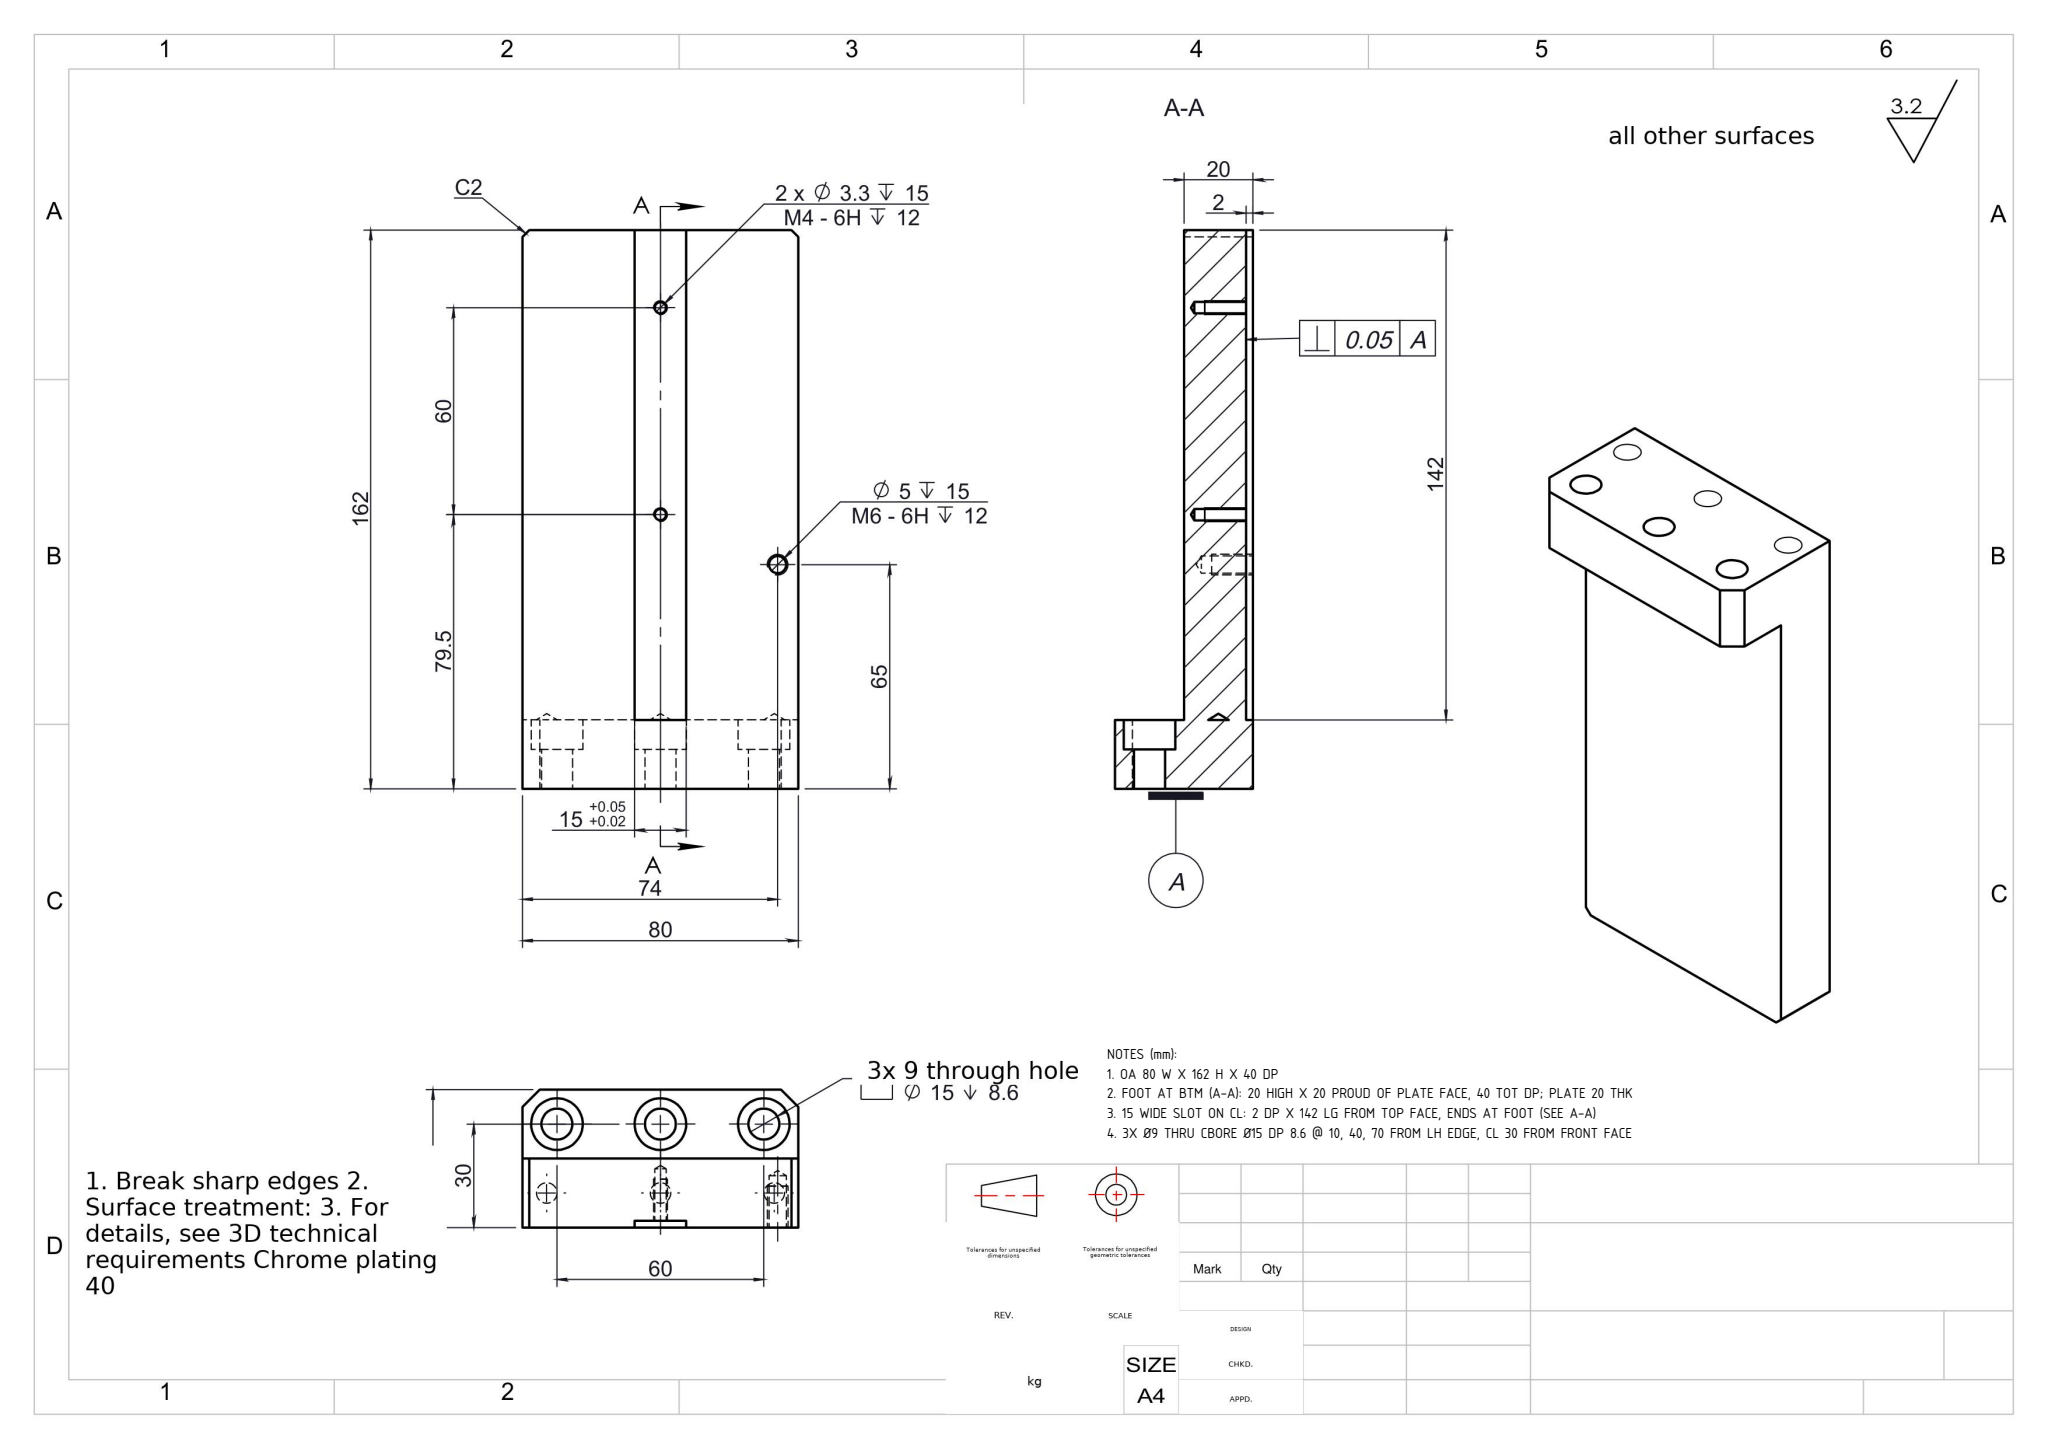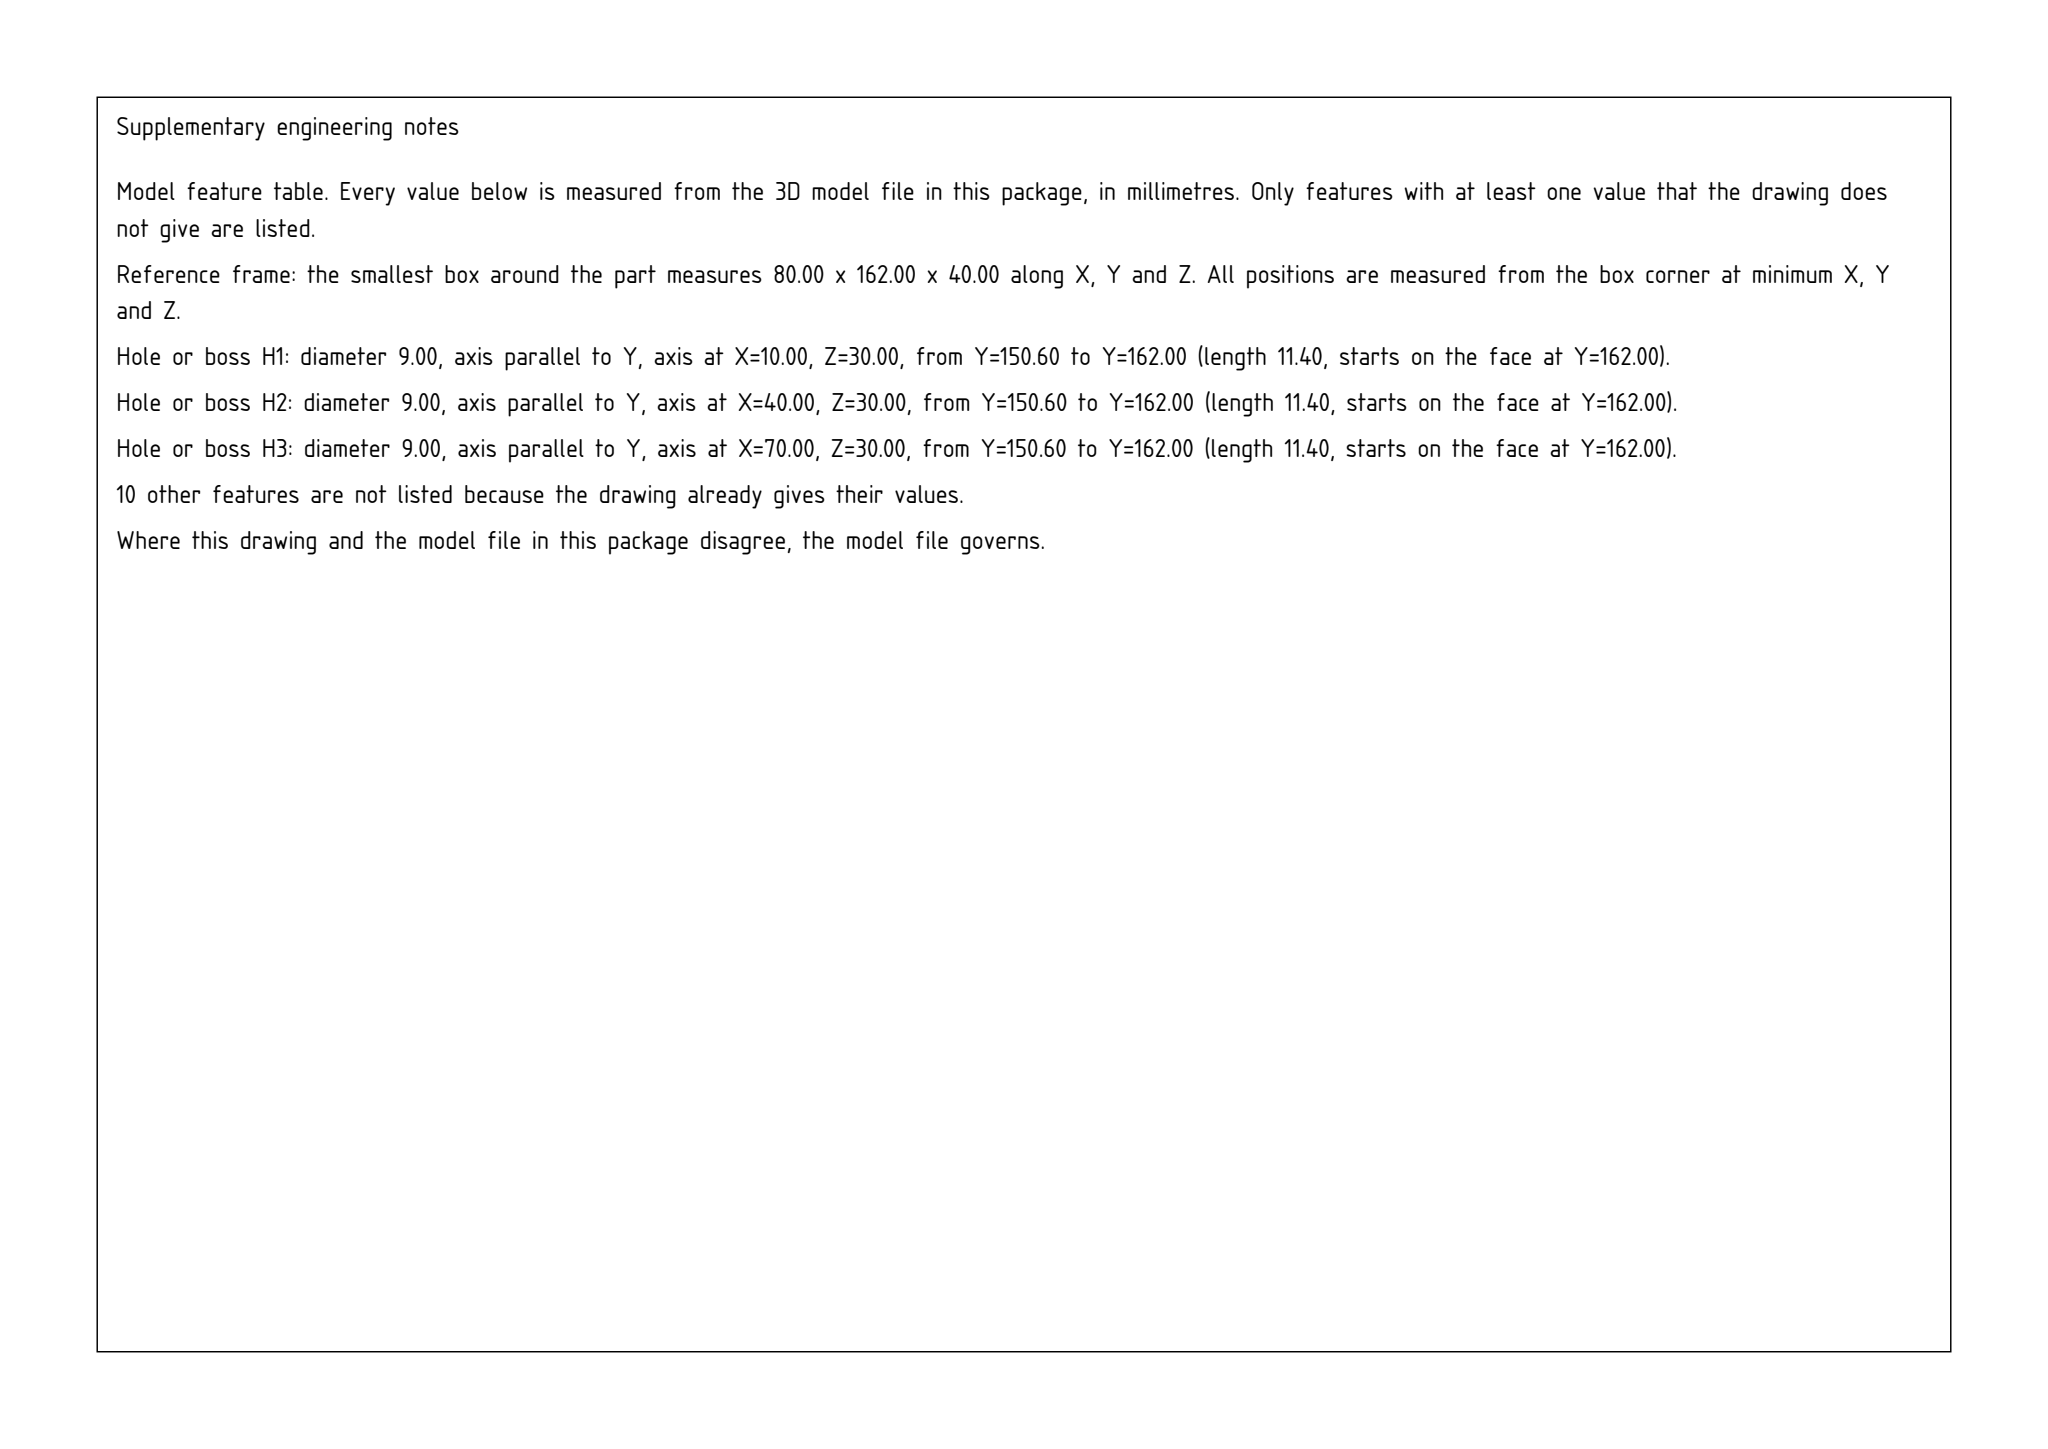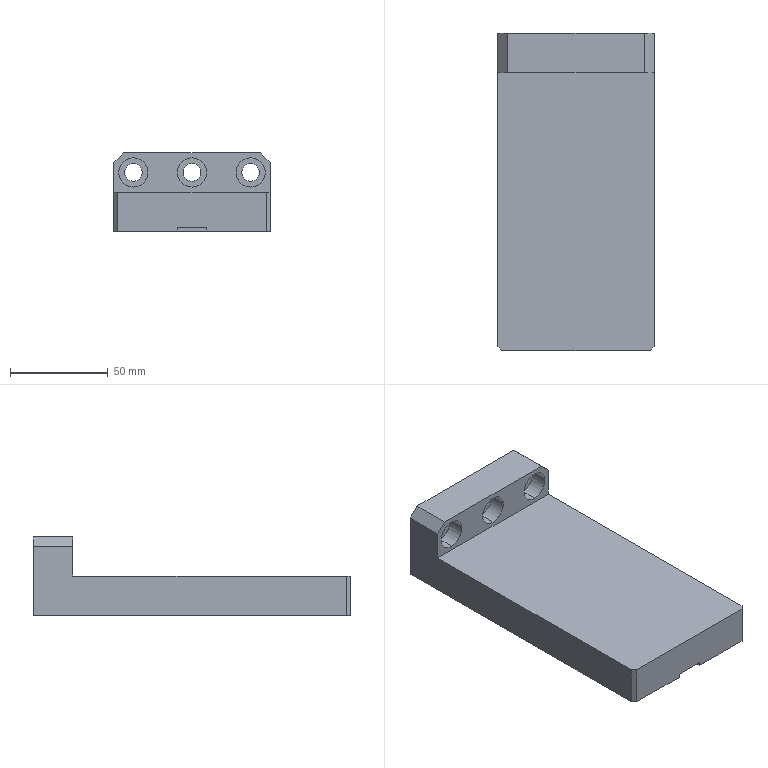Part | SolidWorks | mm | 1 solid | 52 faces | box 80 x 162 x 40 mm | volume 279008 mm3 | plane 22 | cylinder 18 | cone 12 | commonest cylinder face diameters 15 x6 9 x6 3.3 x4 5 x2
Drawing notes:
OA 80 W X 162 H X 40 DP | from the solid: bbox_xyz 80 x 162 x 40
FOOT AT BTM (A-A): 20 HIGH X 20 PROUD OF PLATE FACE, 40 TOT DP; PLATE 20 THK | from the solid: y planes 142 & 162 = 20 high; z planes 0/20/40: plate 20 thk, foot 40 deep
15 WIDE SLOT ON CL: 2 DP X 142 LG FROM TOP FACE, ENDS AT FOOT (SEE A-A) | from the solid: x planes 32.5/47.5 (15 wide, ctr x=40); z planes 0 & 2 (2 DP); slot end face y=142
3X Ø9 THRU CBORE Ø15 DP 8.6 @ 10, 40, 70 FROM LH EDGE, CL 30 FROM FRONT FACE | from the solid: Ø9 y-axis x=10/40/70, z=30, L=11.4 (y150.6-162); Ø15 y-axis L=8.6 (y142-150.6)